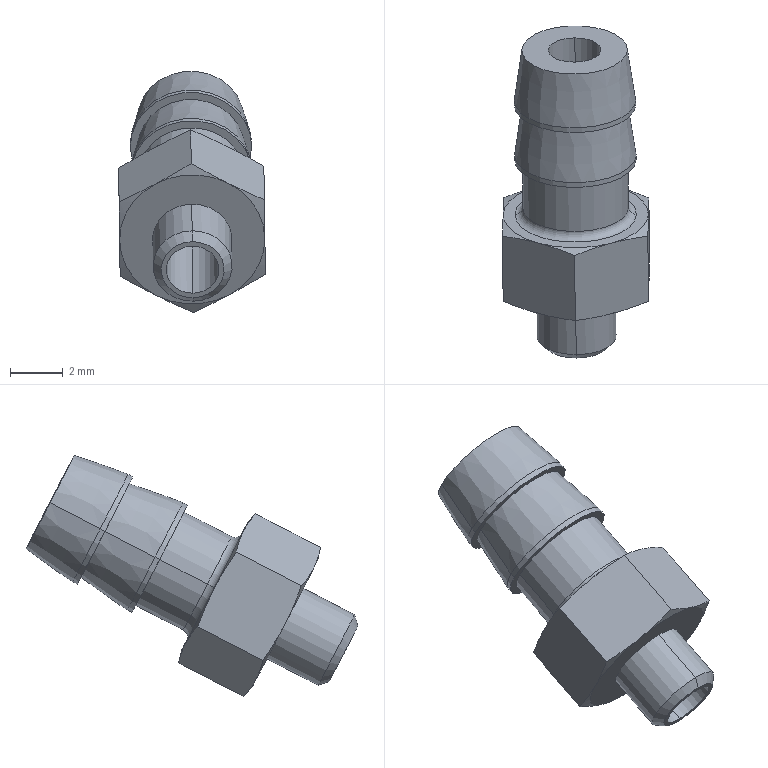Component | SolidWorks | PurchasedPart_MiniConnector03-_4-1 | 1 solid | 42 faces | volume 155 mm3 | cone 18 | plane 12 | cylinder 10 | torus 2 | commonest cylinder face diameters 4.6 x4 2 x2 3 x2 4 x2